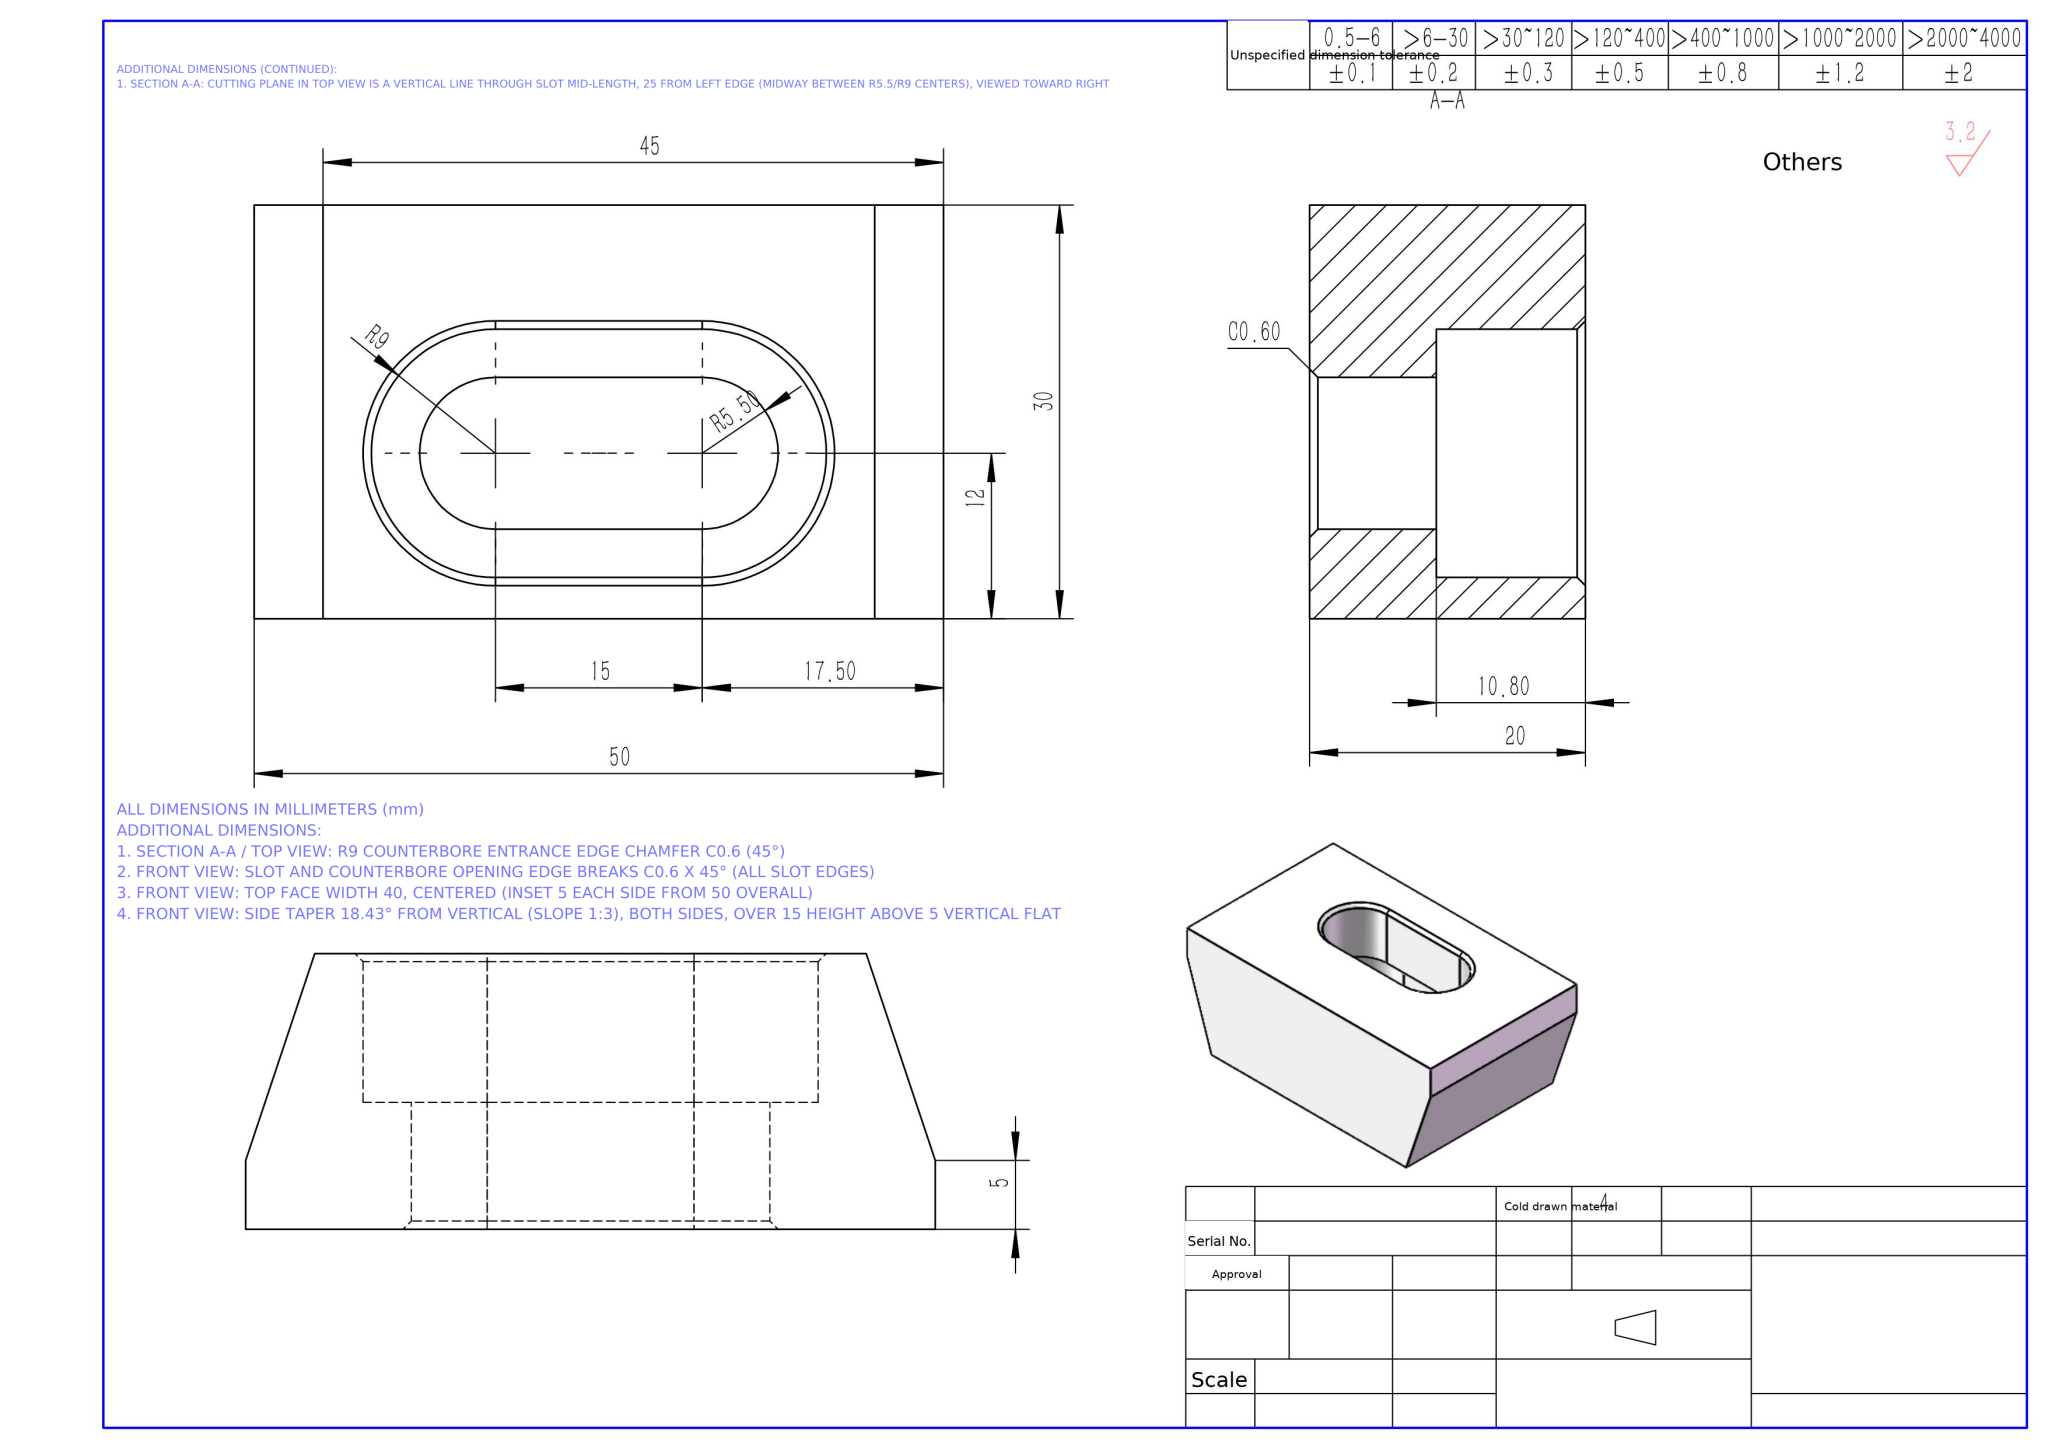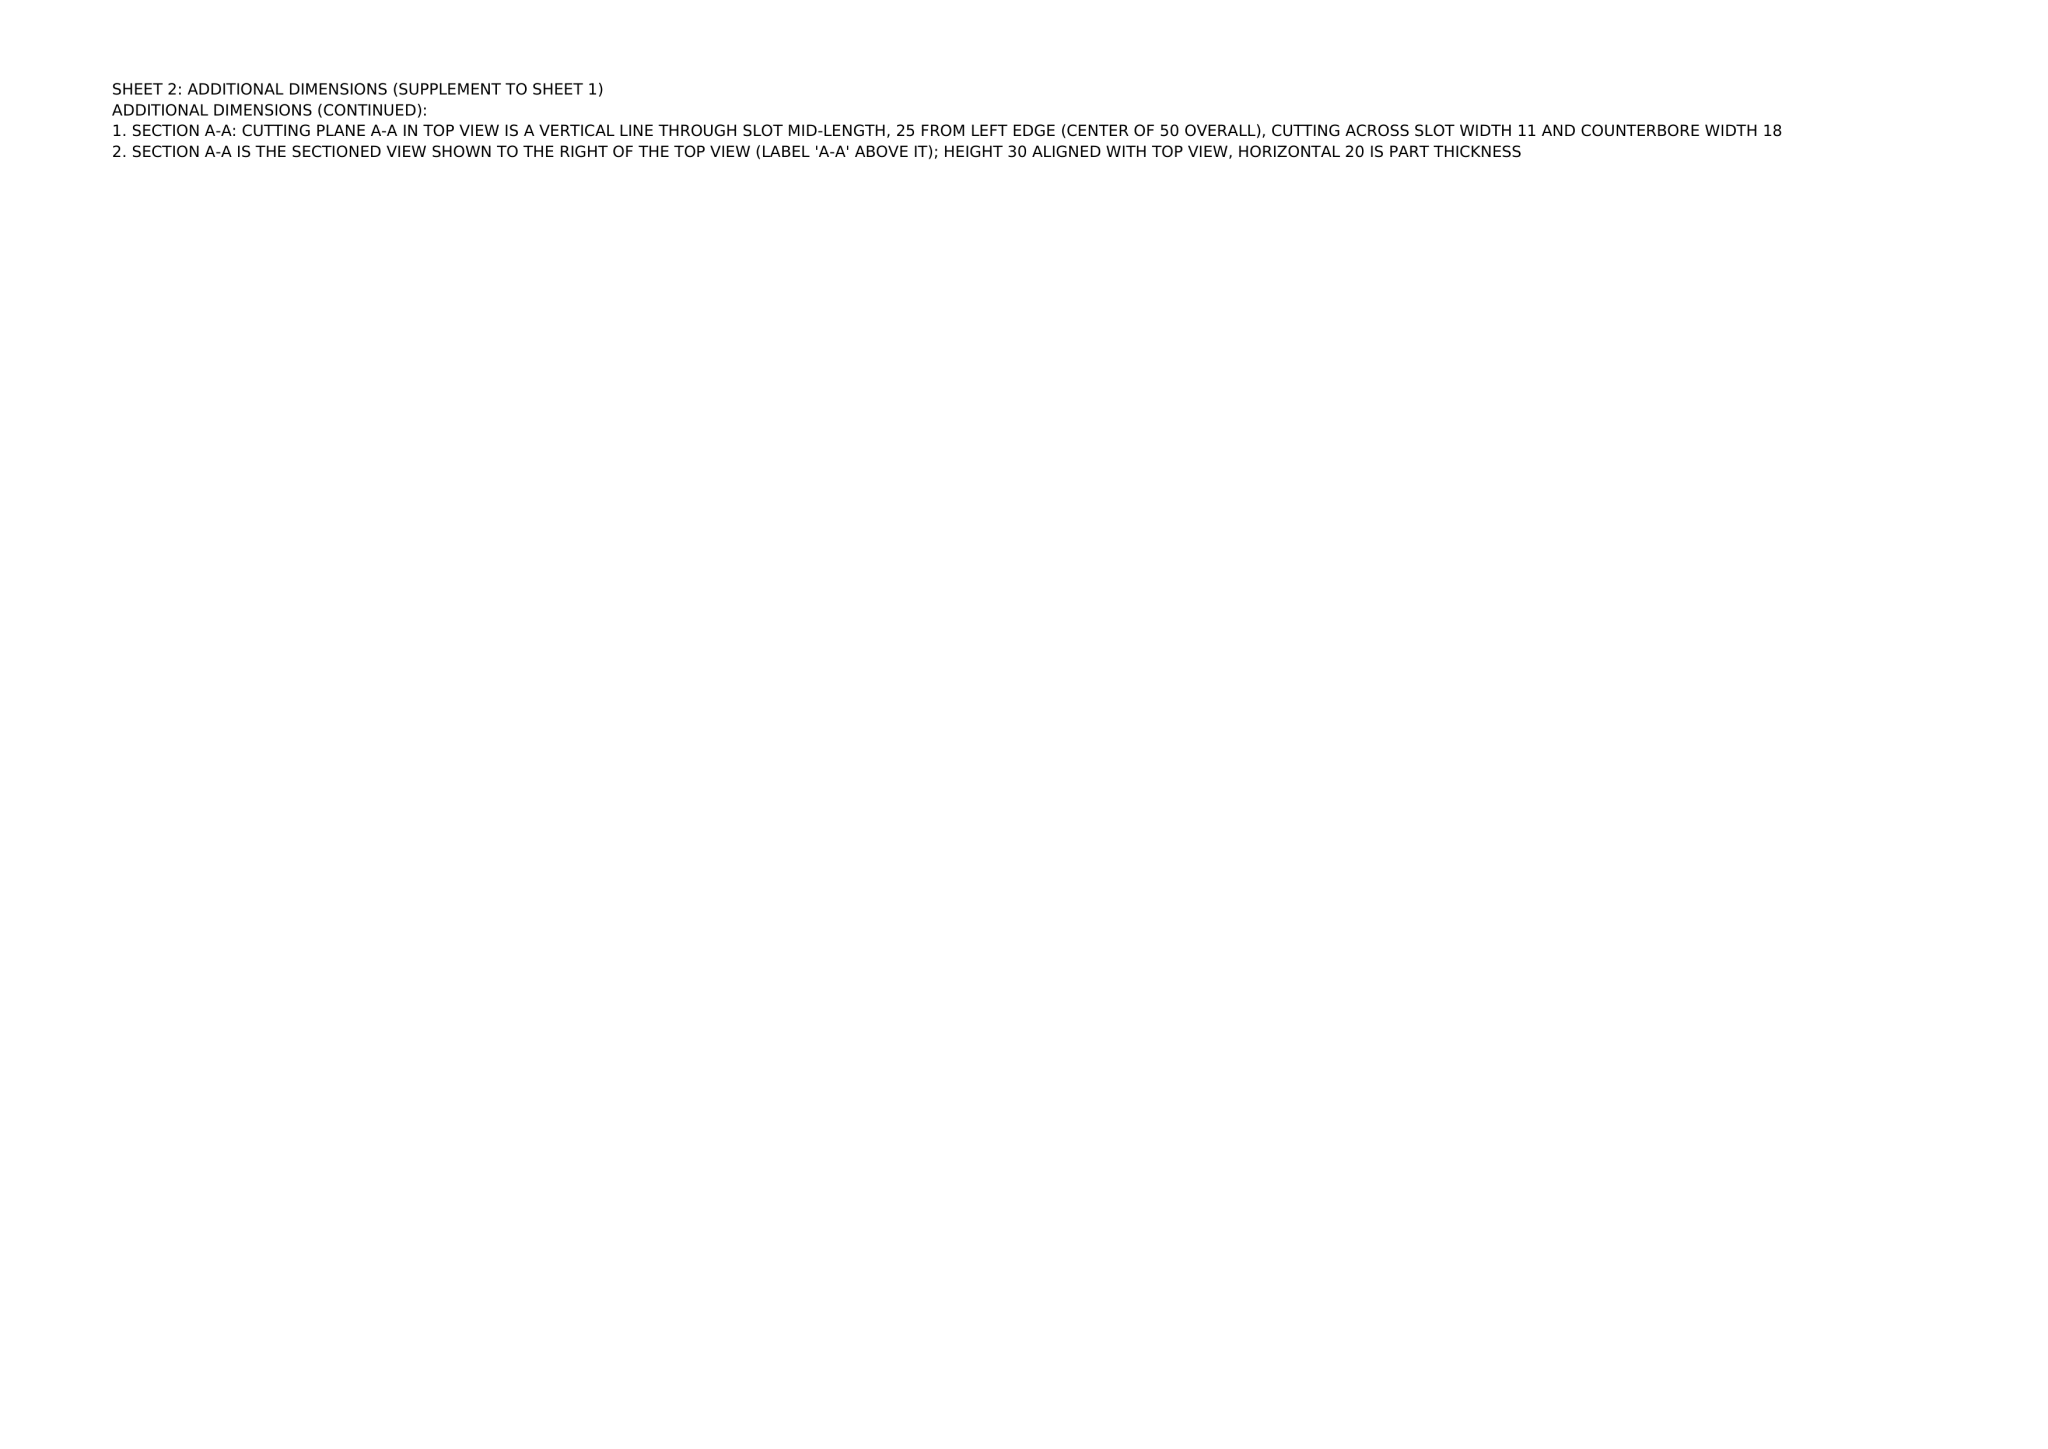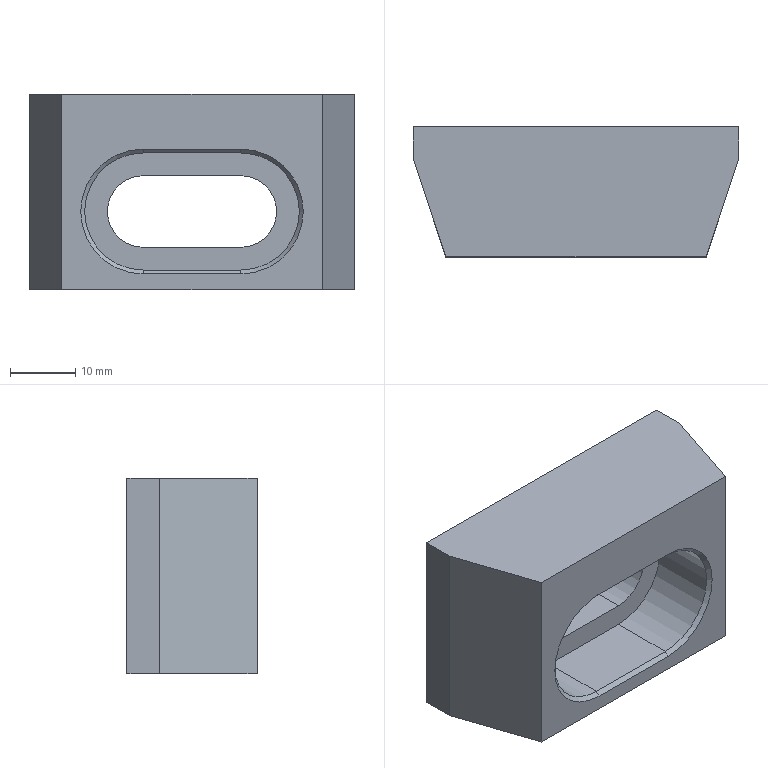Part | NX | mm | 1 solid | 25 faces | box 50 x 20 x 30 mm | volume 19666 mm3 | plane 17 | cone 4 | cylinder 4 | commonest cylinder face diameters 11 x2 18 x2
STEP:
#1=COLOUR_RGB('',1.,1.,1.);
#2=FILL_AREA_STYLE_COLOUR('',#1);
#3=FILL_AREA_STYLE('',(#2));
#4=SURFACE_STYLE_FILL_AREA(#3);
#5=SURFACE_SIDE_STYLE('',(#4));
#6=SURFACE_STYLE_USAGE(.BOTH.,#5);
#7=PRESENTATION_STYLE_ASSIGNMENT((#6));
#8=CARTESIAN_POINT('',(-17.5,-185.8,-4.61));
#9=VERTEX_POINT('',#8);
#10=CARTESIAN_POINT('',(-17.5,-185.8,-16.81));
#11=VERTEX_POINT('',#10);
#12=CARTESIAN_POINT('',(-17.5,-185.8,-10.71));
#13=DIRECTION('',(0.,1.,0.));
#14=DIRECTION('',(0.,0.,1.));
#15=AXIS2_PLACEMENT_3D('',#12,#13,#14);
#16=CIRCLE('',#15,6.1);
#17=EDGE_CURVE('',#9,#11,#16,.T.);
#18=ORIENTED_EDGE('',*,*,#17,.F.);
#19=CARTESIAN_POINT('',(-32.5,-185.8,-4.61));
#20=VERTEX_POINT('',#19);
#21=CARTESIAN_POINT('',(-50.,-185.8,-4.61));
#22=DIRECTION('',(1.,0.,0.));
#23=VECTOR('',#22,1000.);
#24=LINE('',#21,#23);
#25=EDGE_CURVE('',#20,#9,#24,.T.);
#26=ORIENTED_EDGE('',*,*,#25,.F.);
#27=CARTESIAN_POINT('',(-32.5,-185.8,-16.81));
#28=VERTEX_POINT('',#27);
#29=CARTESIAN_POINT('',(-32.5,-185.8,-10.71));
#30=DIRECTION('',(0.,1.,0.));
#31=DIRECTION('',(0.,0.,1.));
#32=AXIS2_PLACEMENT_3D('',#29,#30,#31);
#33=CIRCLE('',#32,6.1);
#34=EDGE_CURVE('',#28,#20,#33,.T.);
#35=ORIENTED_EDGE('',*,*,#34,.F.);
#36=CARTESIAN_POINT('',(-50.,-185.8,-16.81));
#37=DIRECTION('',(-1.,0.,0.));
#38=VECTOR('',#37,1000.);
#39=LINE('',#36,#38);
#40=EDGE_CURVE('',#11,#28,#39,.T.);
#41=ORIENTED_EDGE('',*,*,#40,.F.);
#42=EDGE_LOOP('',(#18,#26,#35,#41));
#43=FACE_BOUND('',#42,.T.);
#44=CARTESIAN_POINT('',(0.,-185.8,-22.71));
#45=VERTEX_POINT('',#44);
#46=CARTESIAN_POINT('',(0.,-185.8,7.29));
#47=VERTEX_POINT('',#46);
#48=CARTESIAN_POINT('',(0.,-185.8,-22.71));
#49=DIRECTION('',(0.,0.,1.));
#50=VECTOR('',#49,1000.);
#51=LINE('',#48,#50);
#52=EDGE_CURVE('',#45,#47,#51,.T.);
#53=ORIENTED_EDGE('',*,*,#52,.F.);
#54=CARTESIAN_POINT('',(-50.,-185.8,-22.71));
#55=VERTEX_POINT('',#54);
#56=CARTESIAN_POINT('',(-50.,-185.8,-22.71));
#57=DIRECTION('',(1.,0.,0.));
#58=VECTOR('',#57,1000.);
#59=LINE('',#56,#58);
#60=EDGE_CURVE('',#55,#45,#59,.T.);
#61=ORIENTED_EDGE('',*,*,#60,.F.);
#62=CARTESIAN_POINT('',(-50.,-185.8,7.29));
#63=VERTEX_POINT('',#62);
#64=CARTESIAN_POINT('',(-50.,-185.8,-22.71));
#65=DIRECTION('',(0.,0.,-1.));
#66=VECTOR('',#65,1000.);
#67=LINE('',#64,#66);
#68=EDGE_CURVE('',#63,#55,#67,.T.);
#69=ORIENTED_EDGE('',*,*,#68,.F.);
#70=CARTESIAN_POINT('',(-50.,-185.8,7.29));
#71=DIRECTION('',(-1.,0.,0.));
#72=VECTOR('',#71,1000.);
#73=LINE('',#70,#72);
#74=EDGE_CURVE('',#47,#63,#73,.T.);
#75=ORIENTED_EDGE('',*,*,#74,.F.);
#76=EDGE_LOOP('',(#53,#61,#69,#75));
#77=FACE_OUTER_BOUND('',#76,.T.);
#78=CARTESIAN_POINT('',(-50.,-185.8,-22.71));
#79=DIRECTION('',(0.,-1.,0.));
#80=DIRECTION('',(0.,0.,-1.));
#81=AXIS2_PLACEMENT_3D('',#78,#79,#80);
#82=PLANE('',#81);
#83=ADVANCED_FACE('',(#43,#77),#82,.F.);
#84=ORIENTED_EDGE('',*,*,#40,.T.);
#85=CARTESIAN_POINT('',(-32.5,-186.4,-16.21));
#86=VERTEX_POINT('',#85);
#87=CARTESIAN_POINT('',(-32.5,-185.8,-16.81));
#88=DIRECTION('',(0.,0.7071,-0.7071));
#89=VECTOR('',#88,1000.);
#90=LINE('',#87,#89);
#91=EDGE_CURVE('',#86,#28,#90,.T.);
#92=ORIENTED_EDGE('',*,*,#91,.F.);
#93=CARTESIAN_POINT('',(-17.5,-186.4,-16.21));
#94=VERTEX_POINT('',#93);
#95=CARTESIAN_POINT('',(-17.5,-186.4,-16.21));
#96=DIRECTION('',(-1.,0.,0.));
#97=VECTOR('',#96,1000.);
#98=LINE('',#95,#97);
#99=EDGE_CURVE('',#94,#86,#98,.T.);
#100=ORIENTED_EDGE('',*,*,#99,.F.);
#101=CARTESIAN_POINT('',(-17.5,-185.8,-16.81));
#102=DIRECTION('',(0.,-0.7071,0.7071));
#103=VECTOR('',#102,1000.);
#104=LINE('',#101,#103);
#105=EDGE_CURVE('',#11,#94,#104,.T.);
#106=ORIENTED_EDGE('',*,*,#105,.F.);
#107=EDGE_LOOP('',(#84,#92,#100,#106));
#108=FACE_OUTER_BOUND('',#107,.T.);
#109=CARTESIAN_POINT('',(-17.5,-185.8,-16.81));
#110=DIRECTION('',(0.,-0.7071,-0.7071));
#111=DIRECTION('',(0.,0.7071,-0.7071));
#112=AXIS2_PLACEMENT_3D('',#109,#110,#111);
#113=PLANE('',#112);
#114=ADVANCED_FACE('',(#108),#113,.F.);
#115=ORIENTED_EDGE('',*,*,#17,.T.);
#116=ORIENTED_EDGE('',*,*,#105,.T.);
#117=CARTESIAN_POINT('',(-17.5,-186.4,-5.21));
#118=VERTEX_POINT('',#117);
#119=CARTESIAN_POINT('',(-17.5,-186.4,-10.71));
#120=DIRECTION('',(0.,1.,0.));
#121=DIRECTION('',(0.,0.,1.));
#122=AXIS2_PLACEMENT_3D('',#119,#120,#121);
#123=CIRCLE('',#122,5.5);
#124=EDGE_CURVE('',#118,#94,#123,.T.);
#125=ORIENTED_EDGE('',*,*,#124,.F.);
#126=CARTESIAN_POINT('',(-17.5,498818.81,499000.));
#127=DIRECTION('',(0.,-0.7071,-0.7071));
#128=VECTOR('',#127,1000.);
#129=LINE('',#126,#128);
#130=EDGE_CURVE('',#9,#118,#129,.T.);
#131=ORIENTED_EDGE('',*,*,#130,.F.);
#132=EDGE_LOOP('',(#115,#116,#125,#131));
#133=FACE_OUTER_BOUND('',#132,.T.);
#134=CARTESIAN_POINT('',(-17.5,-185.8,-10.71));
#135=DIRECTION('',(0.,1.,0.));
#136=DIRECTION('',(0.,0.,1.));
#137=AXIS2_PLACEMENT_3D('',#134,#135,#136);
#138=CONICAL_SURFACE('',#137,6.1,0.7854);
#139=ADVANCED_FACE('',(#133),#138,.F.);
#140=ORIENTED_EDGE('',*,*,#25,.T.);
#141=ORIENTED_EDGE('',*,*,#130,.T.);
#142=CARTESIAN_POINT('',(-32.5,-186.4,-5.21));
#143=VERTEX_POINT('',#142);
#144=CARTESIAN_POINT('',(-17.5,-186.4,-5.21));
#145=DIRECTION('',(1.,0.,0.));
#146=VECTOR('',#145,1000.);
#147=LINE('',#144,#146);
#148=EDGE_CURVE('',#143,#118,#147,.T.);
#149=ORIENTED_EDGE('',*,*,#148,.F.);
#150=CARTESIAN_POINT('',(-32.5,-186.4,-5.21));
#151=DIRECTION('',(0.,-0.7071,-0.7071));
#152=VECTOR('',#151,1000.);
#153=LINE('',#150,#152);
#154=EDGE_CURVE('',#20,#143,#153,.T.);
#155=ORIENTED_EDGE('',*,*,#154,.F.);
#156=EDGE_LOOP('',(#140,#141,#149,#155));
#157=FACE_OUTER_BOUND('',#156,.T.);
#158=CARTESIAN_POINT('',(-17.5,-186.4,-5.21));
#159=DIRECTION('',(0.,-0.7071,0.7071));
#160=DIRECTION('',(0.,-0.7071,-0.7071));
#161=AXIS2_PLACEMENT_3D('',#158,#159,#160);
#162=PLANE('',#161);
#163=ADVANCED_FACE('',(#157),#162,.F.);
#164=ORIENTED_EDGE('',*,*,#154,.T.);
#165=CARTESIAN_POINT('',(-32.5,-186.4,-10.71));
#166=DIRECTION('',(0.,1.,0.));
#167=DIRECTION('',(0.,0.,1.));
#168=AXIS2_PLACEMENT_3D('',#165,#166,#167);
#169=CIRCLE('',#168,5.5);
#170=EDGE_CURVE('',#86,#143,#169,.T.);
#171=ORIENTED_EDGE('',*,*,#170,.F.);
#172=ORIENTED_EDGE('',*,*,#91,.T.);
#173=ORIENTED_EDGE('',*,*,#34,.T.);
#174=EDGE_LOOP('',(#164,#171,#172,#173));
#175=FACE_OUTER_BOUND('',#174,.T.);
#176=CARTESIAN_POINT('',(-32.5,-185.8,-10.71));
#177=DIRECTION('',(0.,1.,0.));
#178=DIRECTION('',(0.,0.,1.));
#179=AXIS2_PLACEMENT_3D('',#176,#177,#178);
#180=CONICAL_SURFACE('',#179,6.1,0.7854);
#181=ADVANCED_FACE('',(#175),#180,.F.);
#182=CARTESIAN_POINT('',(-5.,-205.8,7.29));
#183=VERTEX_POINT('',#182);
#184=CARTESIAN_POINT('',(-45.,-205.8,7.29));
#185=VERTEX_POINT('',#184);
#186=CARTESIAN_POINT('',(0.,-205.8,7.29));
#187=DIRECTION('',(-1.,0.,0.));
#188=VECTOR('',#187,1000.);
#189=LINE('',#186,#188);
#190=EDGE_CURVE('',#183,#185,#189,.T.);
#191=ORIENTED_EDGE('',*,*,#190,.F.);
#192=CARTESIAN_POINT('',(-0.,-190.8,7.29));
#193=VERTEX_POINT('',#192);
#194=CARTESIAN_POINT('',(0.,-190.8,7.29));
#195=DIRECTION('',(-0.3162,-0.9487,0.));
#196=VECTOR('',#195,1000.);
#197=LINE('',#194,#196);
#198=EDGE_CURVE('',#193,#183,#197,.T.);
#199=ORIENTED_EDGE('',*,*,#198,.F.);
#200=CARTESIAN_POINT('',(0.,-205.8,7.29));
#201=DIRECTION('',(0.,-1.,0.));
#202=VECTOR('',#201,1000.);
#203=LINE('',#200,#202);
#204=EDGE_CURVE('',#47,#193,#203,.T.);
#205=ORIENTED_EDGE('',*,*,#204,.F.);
#206=ORIENTED_EDGE('',*,*,#74,.T.);
#207=CARTESIAN_POINT('',(-50.,-190.8,7.29));
#208=VERTEX_POINT('',#207);
#209=CARTESIAN_POINT('',(-50.,-205.8,7.29));
#210=DIRECTION('',(0.,1.,0.));
#211=VECTOR('',#210,1000.);
#212=LINE('',#209,#211);
#213=EDGE_CURVE('',#208,#63,#212,.T.);
#214=ORIENTED_EDGE('',*,*,#213,.F.);
#215=CARTESIAN_POINT('',(-45.,-205.8,7.29));
#216=DIRECTION('',(-0.3162,0.9487,0.));
#217=VECTOR('',#216,1000.);
#218=LINE('',#215,#217);
#219=EDGE_CURVE('',#185,#208,#218,.T.);
#220=ORIENTED_EDGE('',*,*,#219,.F.);
#221=EDGE_LOOP('',(#191,#199,#205,#206,#214,#220));
#222=FACE_OUTER_BOUND('',#221,.T.);
#223=CARTESIAN_POINT('',(0.,-205.8,7.29));
#224=DIRECTION('',(0.,0.,-1.));
#225=DIRECTION('',(-1.,0.,0.));
#226=AXIS2_PLACEMENT_3D('',#223,#224,#225);
#227=PLANE('',#226);
#228=ADVANCED_FACE('',(#222),#227,.F.);
#229=CARTESIAN_POINT('',(-0.,-190.8,-22.71));
#230=VERTEX_POINT('',#229);
#231=CARTESIAN_POINT('',(0.,-205.8,-22.71));
#232=DIRECTION('',(0.,-1.,0.));
#233=VECTOR('',#232,1000.);
#234=LINE('',#231,#233);
#235=EDGE_CURVE('',#45,#230,#234,.T.);
#236=ORIENTED_EDGE('',*,*,#235,.F.);
#237=ORIENTED_EDGE('',*,*,#52,.T.);
#238=ORIENTED_EDGE('',*,*,#204,.T.);
#239=CARTESIAN_POINT('',(0.,-190.8,-22.71));
#240=DIRECTION('',(0.,0.,1.));
#241=VECTOR('',#240,1000.);
#242=LINE('',#239,#241);
#243=EDGE_CURVE('',#230,#193,#242,.T.);
#244=ORIENTED_EDGE('',*,*,#243,.F.);
#245=EDGE_LOOP('',(#236,#237,#238,#244));
#246=FACE_OUTER_BOUND('',#245,.T.);
#247=CARTESIAN_POINT('',(0.,-205.8,-22.71));
#248=DIRECTION('',(-1.,0.,0.));
#249=DIRECTION('',(0.,0.,1.));
#250=AXIS2_PLACEMENT_3D('',#247,#248,#249);
#251=PLANE('',#250);
#252=ADVANCED_FACE('',(#246),#251,.F.);
#253=CARTESIAN_POINT('',(-50.,-190.8,-22.71));
#254=VERTEX_POINT('',#253);
#255=CARTESIAN_POINT('',(-50.,-205.8,-22.71));
#256=DIRECTION('',(0.,-1.,0.));
#257=VECTOR('',#256,1000.);
#258=LINE('',#255,#257);
#259=EDGE_CURVE('',#55,#254,#258,.T.);
#260=ORIENTED_EDGE('',*,*,#259,.F.);
#261=ORIENTED_EDGE('',*,*,#60,.T.);
#262=ORIENTED_EDGE('',*,*,#235,.T.);
#263=CARTESIAN_POINT('',(-5.,-205.8,-22.71));
#264=VERTEX_POINT('',#263);
#265=CARTESIAN_POINT('',(-5.,-205.8,-22.71));
#266=DIRECTION('',(0.3162,0.9487,0.));
#267=VECTOR('',#266,1000.);
#268=LINE('',#265,#267);
#269=EDGE_CURVE('',#264,#230,#268,.T.);
#270=ORIENTED_EDGE('',*,*,#269,.F.);
#271=CARTESIAN_POINT('',(-45.,-205.8,-22.71));
#272=VERTEX_POINT('',#271);
#273=CARTESIAN_POINT('',(-50.,-205.8,-22.71));
#274=DIRECTION('',(1.,0.,0.));
#275=VECTOR('',#274,1000.);
#276=LINE('',#273,#275);
#277=EDGE_CURVE('',#272,#264,#276,.T.);
#278=ORIENTED_EDGE('',*,*,#277,.F.);
#279=CARTESIAN_POINT('',(-50.,-190.8,-22.71));
#280=DIRECTION('',(0.3162,-0.9487,0.));
#281=VECTOR('',#280,1000.);
#282=LINE('',#279,#281);
#283=EDGE_CURVE('',#254,#272,#282,.T.);
#284=ORIENTED_EDGE('',*,*,#283,.F.);
#285=EDGE_LOOP('',(#260,#261,#262,#270,#278,#284));
#286=FACE_OUTER_BOUND('',#285,.T.);
#287=CARTESIAN_POINT('',(-50.,-205.8,-22.71));
#288=DIRECTION('',(0.,0.,1.));
#289=DIRECTION('',(1.,0.,0.));
#290=AXIS2_PLACEMENT_3D('',#287,#288,#289);
#291=PLANE('',#290);
#292=ADVANCED_FACE('',(#286),#291,.F.);
#293=ORIENTED_EDGE('',*,*,#213,.T.);
#294=ORIENTED_EDGE('',*,*,#68,.T.);
#295=ORIENTED_EDGE('',*,*,#259,.T.);
#296=CARTESIAN_POINT('',(-50.,-190.8,7.29));
#297=DIRECTION('',(0.,0.,-1.));
#298=VECTOR('',#297,1000.);
#299=LINE('',#296,#298);
#300=EDGE_CURVE('',#208,#254,#299,.T.);
#301=ORIENTED_EDGE('',*,*,#300,.F.);
#302=EDGE_LOOP('',(#293,#294,#295,#301));
#303=FACE_OUTER_BOUND('',#302,.T.);
#304=CARTESIAN_POINT('',(-50.,-205.8,7.29));
#305=DIRECTION('',(1.,0.,0.));
#306=DIRECTION('',(0.,0.,-1.));
#307=AXIS2_PLACEMENT_3D('',#304,#305,#306);
#308=PLANE('',#307);
#309=ADVANCED_FACE('',(#303),#308,.F.);
#310=CARTESIAN_POINT('',(-17.5,-195.,-16.21));
#311=VERTEX_POINT('',#310);
#312=CARTESIAN_POINT('',(-32.5,-195.,-16.21));
#313=VERTEX_POINT('',#312);
#314=CARTESIAN_POINT('',(-17.5,-195.,-16.21));
#315=DIRECTION('',(-1.,0.,0.));
#316=VECTOR('',#315,1000.);
#317=LINE('',#314,#316);
#318=EDGE_CURVE('',#311,#313,#317,.T.);
#319=ORIENTED_EDGE('',*,*,#318,.F.);
#320=CARTESIAN_POINT('',(-17.5,-186.4,-16.21));
#321=DIRECTION('',(0.,-1.,0.));
#322=VECTOR('',#321,1000.);
#323=LINE('',#320,#322);
#324=EDGE_CURVE('',#94,#311,#323,.T.);
#325=ORIENTED_EDGE('',*,*,#324,.F.);
#326=ORIENTED_EDGE('',*,*,#99,.T.);
#327=CARTESIAN_POINT('',(-32.5,-186.4,-16.21));
#328=DIRECTION('',(0.,1.,0.));
#329=VECTOR('',#328,1000.);
#330=LINE('',#327,#329);
#331=EDGE_CURVE('',#313,#86,#330,.T.);
#332=ORIENTED_EDGE('',*,*,#331,.F.);
#333=EDGE_LOOP('',(#319,#325,#326,#332));
#334=FACE_OUTER_BOUND('',#333,.T.);
#335=CARTESIAN_POINT('',(-17.5,-186.4,-16.21));
#336=DIRECTION('',(0.,0.,-1.));
#337=DIRECTION('',(-1.,0.,0.));
#338=AXIS2_PLACEMENT_3D('',#335,#336,#337);
#339=PLANE('',#338);
#340=ADVANCED_FACE('',(#334),#339,.F.);
#341=CARTESIAN_POINT('',(-17.5,-195.,-5.21));
#342=VERTEX_POINT('',#341);
#343=CARTESIAN_POINT('',(-17.5,-162.121,-5.21));
#344=DIRECTION('',(0.,-1.,0.));
#345=VECTOR('',#344,1000.);
#346=LINE('',#343,#345);
#347=EDGE_CURVE('',#118,#342,#346,.T.);
#348=ORIENTED_EDGE('',*,*,#347,.F.);
#349=ORIENTED_EDGE('',*,*,#124,.T.);
#350=ORIENTED_EDGE('',*,*,#324,.T.);
#351=CARTESIAN_POINT('',(-17.5,-195.,-10.71));
#352=DIRECTION('',(0.,1.,0.));
#353=DIRECTION('',(0.,0.,1.));
#354=AXIS2_PLACEMENT_3D('',#351,#352,#353);
#355=CIRCLE('',#354,5.5);
#356=EDGE_CURVE('',#342,#311,#355,.T.);
#357=ORIENTED_EDGE('',*,*,#356,.F.);
#358=EDGE_LOOP('',(#348,#349,#350,#357));
#359=FACE_OUTER_BOUND('',#358,.T.);
#360=CARTESIAN_POINT('',(-17.5,-162.121,-10.71));
#361=DIRECTION('',(0.,1.,0.));
#362=DIRECTION('',(0.,0.,1.));
#363=AXIS2_PLACEMENT_3D('',#360,#361,#362);
#364=CYLINDRICAL_SURFACE('',#363,5.5);
#365=ADVANCED_FACE('',(#359),#364,.F.);
#366=CARTESIAN_POINT('',(-32.5,-195.,-5.21));
#367=VERTEX_POINT('',#366);
#368=CARTESIAN_POINT('',(-17.5,-195.,-5.21));
#369=DIRECTION('',(1.,0.,0.));
#370=VECTOR('',#369,1000.);
#371=LINE('',#368,#370);
#372=EDGE_CURVE('',#367,#342,#371,.T.);
#373=ORIENTED_EDGE('',*,*,#372,.F.);
#374=CARTESIAN_POINT('',(-32.5,-195.,-5.21));
#375=DIRECTION('',(0.,-1.,0.));
#376=VECTOR('',#375,1000.);
#377=LINE('',#374,#376);
#378=EDGE_CURVE('',#143,#367,#377,.T.);
#379=ORIENTED_EDGE('',*,*,#378,.F.);
#380=ORIENTED_EDGE('',*,*,#148,.T.);
#381=ORIENTED_EDGE('',*,*,#347,.T.);
#382=EDGE_LOOP('',(#373,#379,#380,#381));
#383=FACE_OUTER_BOUND('',#382,.T.);
#384=CARTESIAN_POINT('',(-17.5,-195.,-5.21));
#385=DIRECTION('',(0.,0.,1.));
#386=DIRECTION('',(1.,0.,0.));
#387=AXIS2_PLACEMENT_3D('',#384,#385,#386);
#388=PLANE('',#387);
#389=ADVANCED_FACE('',(#383),#388,.F.);
#390=CARTESIAN_POINT('',(-32.5,-195.,-10.71));
#391=DIRECTION('',(0.,1.,0.));
#392=DIRECTION('',(0.,0.,1.));
#393=AXIS2_PLACEMENT_3D('',#390,#391,#392);
#394=CIRCLE('',#393,5.5);
#395=EDGE_CURVE('',#313,#367,#394,.T.);
#396=ORIENTED_EDGE('',*,*,#395,.F.);
#397=ORIENTED_EDGE('',*,*,#331,.T.);
#398=ORIENTED_EDGE('',*,*,#170,.T.);
#399=ORIENTED_EDGE('',*,*,#378,.T.);
#400=EDGE_LOOP('',(#396,#397,#398,#399));
#401=FACE_OUTER_BOUND('',#400,.T.);
#402=CARTESIAN_POINT('',(-32.5,-162.121,-10.71));
#403=DIRECTION('',(0.,1.,0.));
#404=DIRECTION('',(0.,0.,1.));
#405=AXIS2_PLACEMENT_3D('',#402,#403,#404);
#406=CYLINDRICAL_SURFACE('',#405,5.5);
#407=ADVANCED_FACE('',(#401),#406,.F.);
#408=ORIENTED_EDGE('',*,*,#300,.T.);
#409=ORIENTED_EDGE('',*,*,#283,.T.);
#410=CARTESIAN_POINT('',(-45.,-205.8,7.29));
#411=DIRECTION('',(0.,0.,1.));
#412=VECTOR('',#411,1000.);
#413=LINE('',#410,#412);
#414=EDGE_CURVE('',#272,#185,#413,.T.);
#415=ORIENTED_EDGE('',*,*,#414,.T.);
#416=ORIENTED_EDGE('',*,*,#219,.T.);
#417=EDGE_LOOP('',(#408,#409,#415,#416));
#418=FACE_OUTER_BOUND('',#417,.T.);
#419=CARTESIAN_POINT('',(-50.,-190.8,7.29));
#420=DIRECTION('',(-0.9487,-0.3162,0.));
#421=DIRECTION('',(0.3162,-0.9487,0.));
#422=AXIS2_PLACEMENT_3D('',#419,#420,#421);
#423=PLANE('',#422);
#424=ADVANCED_FACE('',(#418),#423,.T.);
#425=CARTESIAN_POINT('',(-32.5,-205.8,-1.11));
#426=VERTEX_POINT('',#425);
#427=CARTESIAN_POINT('',(-17.5,-205.8,-1.11));
#428=VERTEX_POINT('',#427);
#429=CARTESIAN_POINT('',(-50.,-205.8,-1.11));
#430=DIRECTION('',(1.,0.,0.));
#431=VECTOR('',#430,1000.);
#432=LINE('',#429,#431);
#433=EDGE_CURVE('',#426,#428,#432,.T.);
#434=ORIENTED_EDGE('',*,*,#433,.T.);
#435=CARTESIAN_POINT('',(-17.5,-205.8,-20.31));
#436=VERTEX_POINT('',#435);
#437=CARTESIAN_POINT('',(-17.5,-205.8,-10.71));
#438=DIRECTION('',(0.,1.,0.));
#439=DIRECTION('',(0.,0.,-1.));
#440=AXIS2_PLACEMENT_3D('',#437,#438,#439);
#441=CIRCLE('',#440,9.6);
#442=EDGE_CURVE('',#428,#436,#441,.T.);
#443=ORIENTED_EDGE('',*,*,#442,.T.);
#444=CARTESIAN_POINT('',(-32.5,-205.8,-20.31));
#445=VERTEX_POINT('',#444);
#446=CARTESIAN_POINT('',(-50.,-205.8,-20.31));
#447=DIRECTION('',(-1.,0.,0.));
#448=VECTOR('',#447,1000.);
#449=LINE('',#446,#448);
#450=EDGE_CURVE('',#436,#445,#449,.T.);
#451=ORIENTED_EDGE('',*,*,#450,.T.);
#452=CARTESIAN_POINT('',(-32.5,-205.8,-10.71));
#453=DIRECTION('',(0.,1.,0.));
#454=DIRECTION('',(-0.,0.,-1.));
#455=AXIS2_PLACEMENT_3D('',#452,#453,#454);
#456=CIRCLE('',#455,9.6);
#457=EDGE_CURVE('',#445,#426,#456,.T.);
#458=ORIENTED_EDGE('',*,*,#457,.T.);
#459=EDGE_LOOP('',(#434,#443,#451,#458));
#460=FACE_BOUND('',#459,.T.);
#461=CARTESIAN_POINT('',(-5.,-205.8,-22.71));
#462=DIRECTION('',(0.,0.,1.));
#463=VECTOR('',#462,1000.);
#464=LINE('',#461,#463);
#465=EDGE_CURVE('',#264,#183,#464,.T.);
#466=ORIENTED_EDGE('',*,*,#465,.T.);
#467=ORIENTED_EDGE('',*,*,#190,.T.);
#468=ORIENTED_EDGE('',*,*,#414,.F.);
#469=ORIENTED_EDGE('',*,*,#277,.T.);
#470=EDGE_LOOP('',(#466,#467,#468,#469));
#471=FACE_OUTER_BOUND('',#470,.T.);
#472=CARTESIAN_POINT('',(-50.,-205.8,-22.71));
#473=DIRECTION('',(0.,-1.,0.));
#474=DIRECTION('',(0.,0.,-1.));
#475=AXIS2_PLACEMENT_3D('',#472,#473,#474);
#476=PLANE('',#475);
#477=ADVANCED_FACE('',(#460,#471),#476,.T.);
#478=ORIENTED_EDGE('',*,*,#243,.T.);
#479=ORIENTED_EDGE('',*,*,#198,.T.);
#480=ORIENTED_EDGE('',*,*,#465,.F.);
#481=ORIENTED_EDGE('',*,*,#269,.T.);
#482=EDGE_LOOP('',(#478,#479,#480,#481));
#483=FACE_OUTER_BOUND('',#482,.T.);
#484=CARTESIAN_POINT('',(0.,-190.8,-22.71));
#485=DIRECTION('',(0.9487,-0.3162,0.));
#486=DIRECTION('',(0.3162,0.9487,0.));
#487=AXIS2_PLACEMENT_3D('',#484,#485,#486);
#488=PLANE('',#487);
#489=ADVANCED_FACE('',(#483),#488,.T.);
#490=ORIENTED_EDGE('',*,*,#395,.T.);
#491=ORIENTED_EDGE('',*,*,#372,.T.);
#492=ORIENTED_EDGE('',*,*,#356,.T.);
#493=ORIENTED_EDGE('',*,*,#318,.T.);
#494=EDGE_LOOP('',(#490,#491,#492,#493));
#495=FACE_BOUND('',#494,.T.);
#496=CARTESIAN_POINT('',(-17.5,-195.,-19.71));
#497=VERTEX_POINT('',#496);
#498=CARTESIAN_POINT('',(-32.5,-195.,-19.71));
#499=VERTEX_POINT('',#498);
#500=CARTESIAN_POINT('',(-22.5,-195.,-19.71));
#501=DIRECTION('',(-1.,0.,0.));
#502=VECTOR('',#501,1000.);
#503=LINE('',#500,#502);
#504=EDGE_CURVE('',#497,#499,#503,.T.);
#505=ORIENTED_EDGE('',*,*,#504,.F.);
#506=CARTESIAN_POINT('',(-17.5,-195.,-1.71));
#507=VERTEX_POINT('',#506);
#508=CARTESIAN_POINT('',(-17.5,-195.,-10.71));
#509=DIRECTION('',(0.,1.,0.));
#510=DIRECTION('',(0.,0.,1.));
#511=AXIS2_PLACEMENT_3D('',#508,#509,#510);
#512=CIRCLE('',#511,9.);
#513=EDGE_CURVE('',#507,#497,#512,.T.);
#514=ORIENTED_EDGE('',*,*,#513,.F.);
#515=CARTESIAN_POINT('',(-32.5,-195.,-1.71));
#516=VERTEX_POINT('',#515);
#517=CARTESIAN_POINT('',(-22.5,-195.,-1.71));
#518=DIRECTION('',(1.,0.,0.));
#519=VECTOR('',#518,1000.);
#520=LINE('',#517,#519);
#521=EDGE_CURVE('',#516,#507,#520,.T.);
#522=ORIENTED_EDGE('',*,*,#521,.F.);
#523=CARTESIAN_POINT('',(-32.5,-195.,-10.71));
#524=DIRECTION('',(0.,1.,0.));
#525=DIRECTION('',(0.,0.,1.));
#526=AXIS2_PLACEMENT_3D('',#523,#524,#525);
#527=CIRCLE('',#526,9.);
#528=EDGE_CURVE('',#499,#516,#527,.T.);
#529=ORIENTED_EDGE('',*,*,#528,.F.);
#530=EDGE_LOOP('',(#505,#514,#522,#529));
#531=FACE_OUTER_BOUND('',#530,.T.);
#532=CARTESIAN_POINT('',(-22.5,-195.,-10.71));
#533=DIRECTION('',(0.,1.,0.));
#534=DIRECTION('',(0.,0.,1.));
#535=AXIS2_PLACEMENT_3D('',#532,#533,#534);
#536=PLANE('',#535);
#537=ADVANCED_FACE('',(#495,#531),#536,.F.);
#538=ORIENTED_EDGE('',*,*,#442,.F.);
#539=CARTESIAN_POINT('',(-17.5,-205.2,-1.71));
#540=VERTEX_POINT('',#539);
#541=CARTESIAN_POINT('',(-17.5,-205.5,-1.41));
#542=DIRECTION('',(0.,-0.7071,0.7071));
#543=VECTOR('',#542,1000.);
#544=LINE('',#541,#543);
#545=EDGE_CURVE('',#540,#428,#544,.T.);
#546=ORIENTED_EDGE('',*,*,#545,.F.);
#547=CARTESIAN_POINT('',(-17.5,-205.2,-19.71));
#548=VERTEX_POINT('',#547);
#549=CARTESIAN_POINT('',(-17.5,-205.2,-10.71));
#550=DIRECTION('',(0.,-1.,0.));
#551=DIRECTION('',(0.,0.,-1.));
#552=AXIS2_PLACEMENT_3D('',#549,#550,#551);
#553=CIRCLE('',#552,9.);
#554=EDGE_CURVE('',#548,#540,#553,.T.);
#555=ORIENTED_EDGE('',*,*,#554,.F.);
#556=CARTESIAN_POINT('',(-17.5,-205.5,-20.01));
#557=DIRECTION('',(0.,0.7071,0.7071));
#558=VECTOR('',#557,1000.);
#559=LINE('',#556,#558);
#560=EDGE_CURVE('',#436,#548,#559,.T.);
#561=ORIENTED_EDGE('',*,*,#560,.F.);
#562=EDGE_LOOP('',(#538,#546,#555,#561));
#563=FACE_OUTER_BOUND('',#562,.T.);
#564=CARTESIAN_POINT('',(-17.5,-205.8,-10.71));
#565=DIRECTION('',(0.,-1.,0.));
#566=DIRECTION('',(0.,0.,-1.));
#567=AXIS2_PLACEMENT_3D('',#564,#565,#566);
#568=CONICAL_SURFACE('',#567,9.6,0.7854);
#569=ADVANCED_FACE('',(#563),#568,.F.);
#570=ORIENTED_EDGE('',*,*,#433,.F.);
#571=CARTESIAN_POINT('',(-32.5,-205.2,-1.71));
#572=VERTEX_POINT('',#571);
#573=CARTESIAN_POINT('',(-32.5,-205.8,-1.11));
#574=DIRECTION('',(0.,-0.7071,0.7071));
#575=VECTOR('',#574,1000.);
#576=LINE('',#573,#575);
#577=EDGE_CURVE('',#572,#426,#576,.T.);
#578=ORIENTED_EDGE('',*,*,#577,.F.);
#579=CARTESIAN_POINT('',(-17.5,-205.2,-1.71));
#580=DIRECTION('',(-1.,0.,0.));
#581=VECTOR('',#580,1000.);
#582=LINE('',#579,#581);
#583=EDGE_CURVE('',#540,#572,#582,.T.);
#584=ORIENTED_EDGE('',*,*,#583,.F.);
#585=ORIENTED_EDGE('',*,*,#545,.T.);
#586=EDGE_LOOP('',(#570,#578,#584,#585));
#587=FACE_OUTER_BOUND('',#586,.T.);
#588=CARTESIAN_POINT('',(-17.5,-205.8,-1.11));
#589=DIRECTION('',(0.,0.7071,0.7071));
#590=DIRECTION('',(0.,-0.7071,0.7071));
#591=AXIS2_PLACEMENT_3D('',#588,#589,#590);
#592=PLANE('',#591);
#593=ADVANCED_FACE('',(#587),#592,.F.);
#594=CARTESIAN_POINT('',(-32.5,-205.2,-19.71));
#595=VERTEX_POINT('',#594);
#596=CARTESIAN_POINT('',(-32.5,-205.5,-20.01));
#597=DIRECTION('',(0.,-0.7071,-0.7071));
#598=VECTOR('',#597,1000.);
#599=LINE('',#596,#598);
#600=EDGE_CURVE('',#595,#445,#599,.T.);
#601=ORIENTED_EDGE('',*,*,#600,.F.);
#602=CARTESIAN_POINT('',(-32.5,-205.2,-10.71));
#603=DIRECTION('',(0.,-1.,0.));
#604=DIRECTION('',(0.,0.,-1.));
#605=AXIS2_PLACEMENT_3D('',#602,#603,#604);
#606=CIRCLE('',#605,9.);
#607=EDGE_CURVE('',#572,#595,#606,.T.);
#608=ORIENTED_EDGE('',*,*,#607,.F.);
#609=ORIENTED_EDGE('',*,*,#577,.T.);
#610=ORIENTED_EDGE('',*,*,#457,.F.);
#611=EDGE_LOOP('',(#601,#608,#609,#610));
#612=FACE_OUTER_BOUND('',#611,.T.);
#613=CARTESIAN_POINT('',(-32.5,-205.8,-10.71));
#614=DIRECTION('',(0.,-1.,0.));
#615=DIRECTION('',(0.,0.,-1.));
#616=AXIS2_PLACEMENT_3D('',#613,#614,#615);
#617=CONICAL_SURFACE('',#616,9.6,0.7854);
#618=ADVANCED_FACE('',(#612),#617,.F.);
#619=ORIENTED_EDGE('',*,*,#450,.F.);
#620=ORIENTED_EDGE('',*,*,#560,.T.);
#621=CARTESIAN_POINT('',(-17.5,-205.2,-19.71));
#622=DIRECTION('',(1.,0.,0.));
#623=VECTOR('',#622,1000.);
#624=LINE('',#621,#623);
#625=EDGE_CURVE('',#595,#548,#624,.T.);
#626=ORIENTED_EDGE('',*,*,#625,.F.);
#627=ORIENTED_EDGE('',*,*,#600,.T.);
#628=EDGE_LOOP('',(#619,#620,#626,#627));
#629=FACE_OUTER_BOUND('',#628,.T.);
#630=CARTESIAN_POINT('',(-17.5,-205.2,-19.71));
#631=DIRECTION('',(0.,0.7071,-0.7071));
#632=DIRECTION('',(0.,0.7071,0.7071));
#633=AXIS2_PLACEMENT_3D('',#630,#631,#632);
#634=PLANE('',#633);
#635=ADVANCED_FACE('',(#629),#634,.F.);
#636=ORIENTED_EDGE('',*,*,#607,.T.);
#637=CARTESIAN_POINT('',(-32.5,-205.8,-19.71));
#638=DIRECTION('',(0.,-1.,0.));
#639=VECTOR('',#638,1000.);
#640=LINE('',#637,#639);
#641=EDGE_CURVE('',#499,#595,#640,.T.);
#642=ORIENTED_EDGE('',*,*,#641,.F.);
#643=ORIENTED_EDGE('',*,*,#528,.T.);
#644=CARTESIAN_POINT('',(-32.5,-205.8,-1.71));
#645=DIRECTION('',(0.,1.,0.));
#646=VECTOR('',#645,1000.);
#647=LINE('',#644,#646);
#648=EDGE_CURVE('',#572,#516,#647,.T.);
#649=ORIENTED_EDGE('',*,*,#648,.F.);
#650=EDGE_LOOP('',(#636,#642,#643,#649));
#651=FACE_OUTER_BOUND('',#650,.T.);
#652=CARTESIAN_POINT('',(-32.5,-205.8,-10.71));
#653=DIRECTION('',(0.,1.,0.));
#654=DIRECTION('',(0.,0.,1.));
#655=AXIS2_PLACEMENT_3D('',#652,#653,#654);
#656=CYLINDRICAL_SURFACE('',#655,9.);
#657=ADVANCED_FACE('',(#651),#656,.F.);
#658=ORIENTED_EDGE('',*,*,#625,.T.);
#659=CARTESIAN_POINT('',(-17.5,-195.,-19.71));
#660=DIRECTION('',(0.,-1.,0.));
#661=VECTOR('',#660,1000.);
#662=LINE('',#659,#661);
#663=EDGE_CURVE('',#497,#548,#662,.T.);
#664=ORIENTED_EDGE('',*,*,#663,.F.);
#665=ORIENTED_EDGE('',*,*,#504,.T.);
#666=ORIENTED_EDGE('',*,*,#641,.T.);
#667=EDGE_LOOP('',(#658,#664,#665,#666));
#668=FACE_OUTER_BOUND('',#667,.T.);
#669=CARTESIAN_POINT('',(-17.5,-195.,-19.71));
#670=DIRECTION('',(0.,0.,-1.));
#671=DIRECTION('',(-1.,0.,0.));
#672=AXIS2_PLACEMENT_3D('',#669,#670,#671);
#673=PLANE('',#672);
#674=ADVANCED_FACE('',(#668),#673,.F.);
#675=CARTESIAN_POINT('',(-17.5,-205.8,-1.71));
#676=DIRECTION('',(0.,-1.,0.));
#677=VECTOR('',#676,1000.);
#678=LINE('',#675,#677);
#679=EDGE_CURVE('',#507,#540,#678,.T.);
#680=ORIENTED_EDGE('',*,*,#679,.F.);
#681=ORIENTED_EDGE('',*,*,#513,.T.);
#682=ORIENTED_EDGE('',*,*,#663,.T.);
#683=ORIENTED_EDGE('',*,*,#554,.T.);
#684=EDGE_LOOP('',(#680,#681,#682,#683));
#685=FACE_OUTER_BOUND('',#684,.T.);
#686=CARTESIAN_POINT('',(-17.5,-205.8,-10.71));
#687=DIRECTION('',(0.,1.,0.));
#688=DIRECTION('',(0.,0.,1.));
#689=AXIS2_PLACEMENT_3D('',#686,#687,#688);
#690=CYLINDRICAL_SURFACE('',#689,9.);
#691=ADVANCED_FACE('',(#685),#690,.F.);
#692=ORIENTED_EDGE('',*,*,#583,.T.);
#693=ORIENTED_EDGE('',*,*,#648,.T.);
#694=ORIENTED_EDGE('',*,*,#521,.T.);
#695=ORIENTED_EDGE('',*,*,#679,.T.);
#696=EDGE_LOOP('',(#692,#693,#694,#695));
#697=FACE_OUTER_BOUND('',#696,.T.);
#698=CARTESIAN_POINT('',(-17.5,-205.2,-1.71));
#699=DIRECTION('',(0.,0.,1.));
#700=DIRECTION('',(1.,0.,0.));
#701=AXIS2_PLACEMENT_3D('',#698,#699,#700);
#702=PLANE('',#701);
#703=ADVANCED_FACE('',(#697),#702,.F.);
#704=CLOSED_SHELL('',(#83,#114,#139,#163,#181,#228,#252,#292,#309,#340,#365,#389,#407,#424,#477,#489,#537,#569,#593,#618,#635,#657,#674,#691,#703));
#705=MANIFOLD_SOLID_BREP('',#704);
#706=CARTESIAN_POINT('',(0.,0.,0.));
#707=DIRECTION('',(0.,0.,1.));
#708=DIRECTION('',(1.,0.,0.));
#709=AXIS2_PLACEMENT_3D('',#706,#707,#708);
#710=(LENGTH_UNIT()NAMED_UNIT(*)SI_UNIT(.MILLI.,.METRE.));
#711=UNCERTAINTY_MEASURE_WITH_UNIT(LENGTH_MEASURE(0.00001),#710,'','');
#712=(NAMED_UNIT(*)PLANE_ANGLE_UNIT()SI_UNIT($,.RADIAN.));
#713=(NAMED_UNIT(*)SI_UNIT($,.STERADIAN.)SOLID_ANGLE_UNIT());
#714=(GEOMETRIC_REPRESENTATION_CONTEXT(3)GLOBAL_UNCERTAINTY_ASSIGNED_CONTEXT((#711))GLOBAL_UNIT_ASSIGNED_CONTEXT((#710,#712,#713))REPRESENTATION_CONTEXT('',''));
#715=ADVANCED_BREP_SHAPE_REPRESENTATION('',(#705,#709),#714);
#716=STYLED_ITEM('',(#7),#715);
#717=(LENGTH_UNIT()NAMED_UNIT(*)SI_UNIT(.MILLI.,.METRE.));
#718=UNCERTAINTY_MEASURE_WITH_UNIT(LENGTH_MEASURE(0.00001),#717,'','');
#719=(NAMED_UNIT(*)PLANE_ANGLE_UNIT()SI_UNIT($,.RADIAN.));
#720=(NAMED_UNIT(*)SI_UNIT($,.STERADIAN.)SOLID_ANGLE_UNIT());
#721=(GEOMETRIC_REPRESENTATION_CONTEXT(3)GLOBAL_UNCERTAINTY_ASSIGNED_CONTEXT((#718))GLOBAL_UNIT_ASSIGNED_CONTEXT((#717,#719,#720))REPRESENTATION_CONTEXT('',''));
#722=MECHANICAL_DESIGN_GEOMETRIC_PRESENTATION_REPRESENTATION('',(#716),#721);
#723=COLOUR_RGB('',1.,1.,1.);
#724=FILL_AREA_STYLE_COLOUR('',#723);
#725=FILL_AREA_STYLE('',(#724));
#726=SURFACE_STYLE_FILL_AREA(#725);
#727=SURFACE_SIDE_STYLE('',(#726));
#728=SURFACE_STYLE_USAGE(.BOTH.,#727);
#729=PRESENTATION_STYLE_ASSIGNMENT((#728));
#730=STYLED_ITEM('',(#729),#705);
#731=PRESENTATION_LAYER_ASSIGNMENT('','',(#730));
#732=PRESENTATION_LAYER_ASSIGNMENT('','',(#716));
#733=(LENGTH_UNIT()NAMED_UNIT(*)SI_UNIT(.MILLI.,.METRE.));
#734=UNCERTAINTY_MEASURE_WITH_UNIT(LENGTH_MEASURE(0.00001),#733,'','');
#735=(NAMED_UNIT(*)PLANE_ANGLE_UNIT()SI_UNIT($,.RADIAN.));
#736=(NAMED_UNIT(*)SI_UNIT($,.STERADIAN.)SOLID_ANGLE_UNIT());
#737=(GEOMETRIC_REPRESENTATION_CONTEXT(3)GLOBAL_UNCERTAINTY_ASSIGNED_CONTEXT((#734))GLOBAL_UNIT_ASSIGNED_CONTEXT((#733,#735,#736))REPRESENTATION_CONTEXT('',''));
#738=MECHANICAL_DESIGN_GEOMETRIC_PRESENTATION_REPRESENTATION('',(#730),#737);